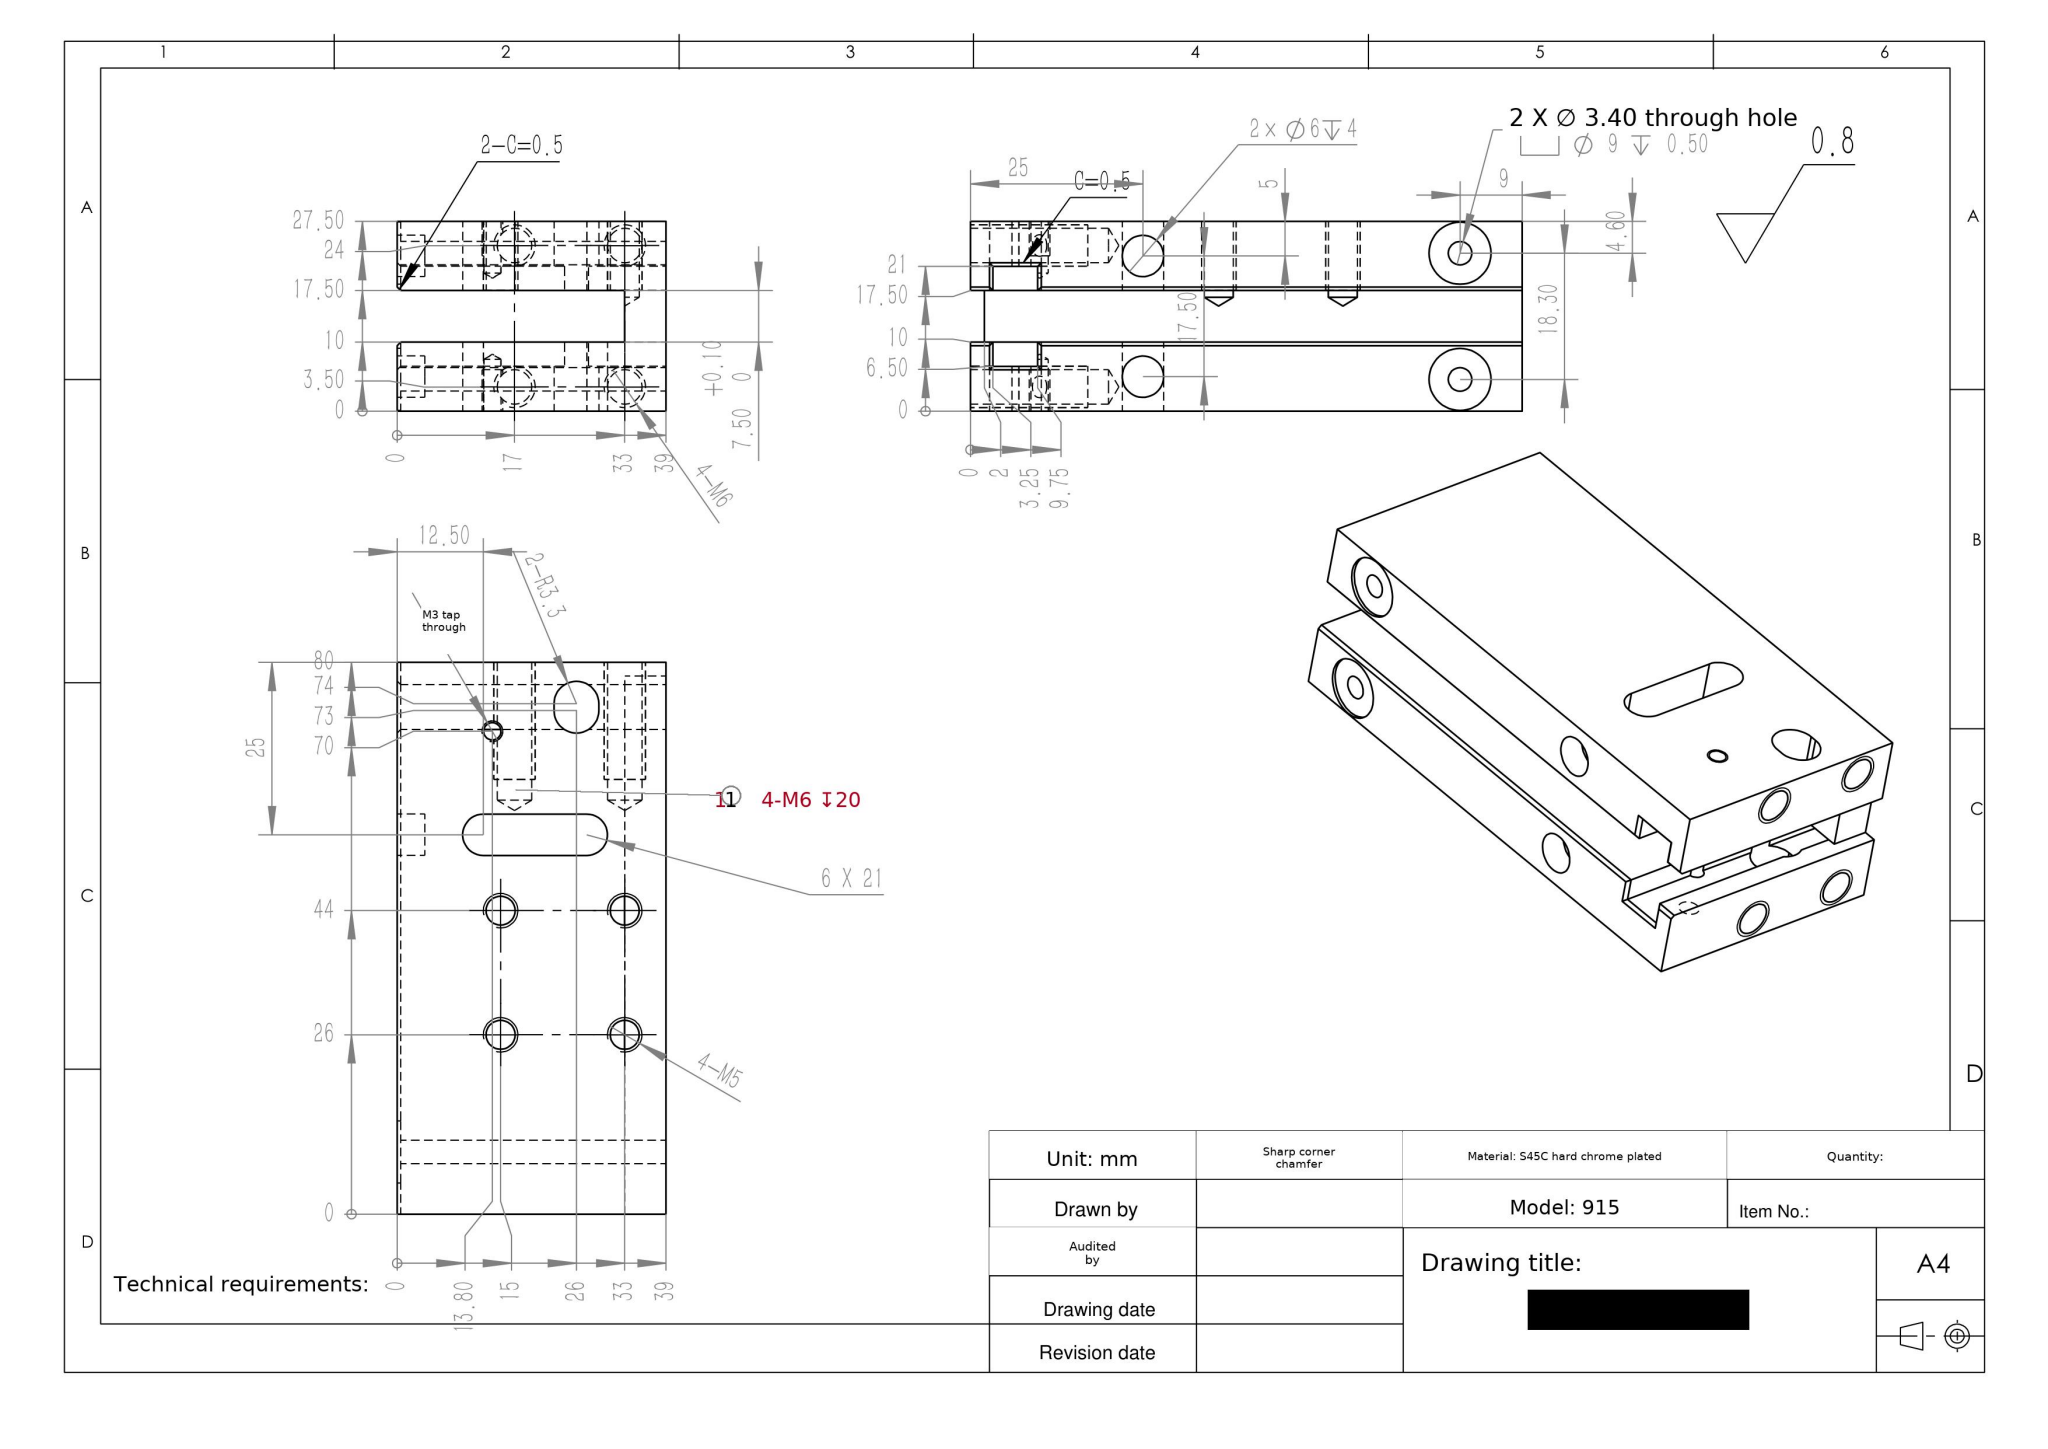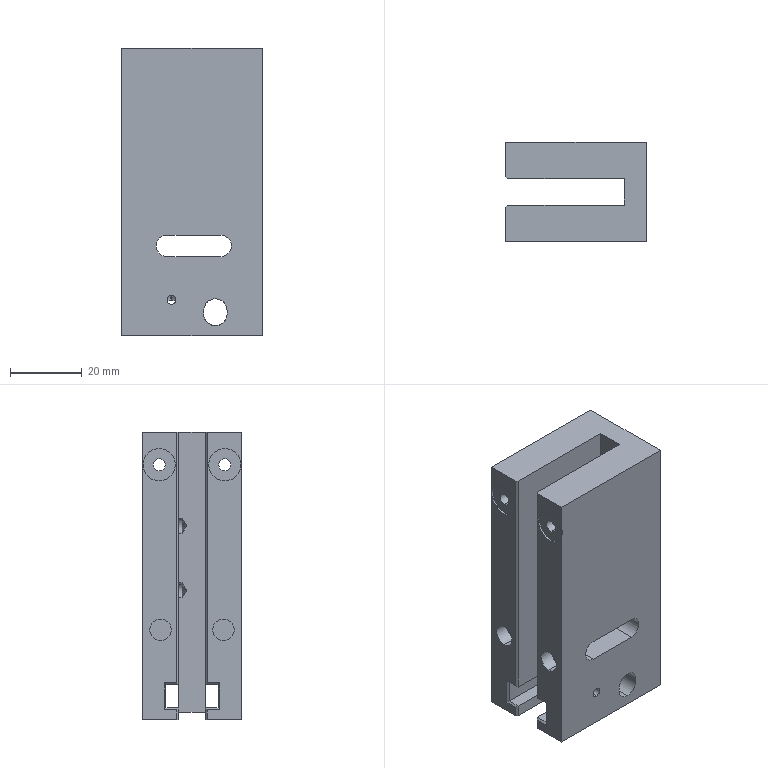Part | SolidWorks | mm | material S45C hard chrome plated | 1 solid | 106 faces | box 39 x 27.5 x 80 mm | volume 57974 mm3 | plane 50 | cylinder 42 | cone 14 | commonest cylinder face diameters 6 x8 5 x8 4.2 x8 6.5 x6 9 x4 3.4 x4 2.5 x4
build123d program:
from build123d import *

# Parameters (mm, degrees)
BOSS_EXTRUDE1_DEPTH                                 = 80
CHAMFER1_SIZE                                       = 0.5
SKETCH3_R                                           = 3.25
CUT_EXTRUDE1_DEPTH                                  = 94.152
SKETCH4_W                                           = 6.5
SKETCH4_H                                           = 3.5
CUT_EXTRUDE2_DEPTH                                  = 94.152
M5_TAPPED_HOLE1_D                                   = 4.2
M5_TAPPED_HOLE1_DEPTH                               = 11
M5_TAPPED_HOLE1_TIP                                 = 1.262
M6_TAPPED_HOLE1_D                                   = 5
M6_TAPPED_HOLE1_DEPTH                               = 20
M6_TAPPED_HOLE1_TIP                                 = 1.502
SKETCH8_W                                           = 6
SKETCH8_H                                           = 7.5
CUT_EXTRUDE3_DEPTH                                  = 2
CHAMFER2_SIZE                                       = 0.5
M3_TAPPED_HOLE1_D                                   = 2.5
M3_TAPPED_HOLE1_DEPTH                               = 7.5
M3_TAPPED_HOLE1_TIP                                 = 0.7511
M3_TAPPED_HOLE2_D                                   = 2.5
M3_TAPPED_HOLE2_DEPTH                               = 7.5
M3_TAPPED_HOLE2_TIP                                 = 0.7511
CUT_EXTRUDE4_DEPTH                                  = 94.152
CUT_EXTRUDE5_DEPTH                                  = 94.152
CYLINDRICAL_COUNTERSUNK_HOLE_FOR_M3_HEX_D           = 3.4
CYLINDRICAL_COUNTERSUNK_HOLE_FOR_M3_HEX_CBORE_D     = 9
CYLINDRICAL_COUNTERSUNK_HOLE_FOR_M3_HEX_CBORE_DEPTH = 0.5
SKETCH18_R                                          = 3
CUT_EXTRUDE6_DEPTH                                  = 4


with BuildPart() as part:
    # Sketch1 → Boss-Extrude1 (new body)
    with BuildSketch(Plane.XY):
        Polygon((0, 17.5), (0, 27.5), (39, 27.5), (39, 0), (0, 0), (0, 10), (33, 10), (33, 17.5), align=None)
    extrude(amount=BOSS_EXTRUDE1_DEPTH)

    # Chamfer1
    chamfer1_edges = [part.edges().sort_by_distance(p)[0] for p in [
        (0, 10, 40),
        (0, 17.5, 40),
    ]]
    chamfer(chamfer1_edges, length=CHAMFER1_SIZE)

    # Sketch3 → Cut-Extrude1 (cut, through all)
    with BuildSketch(Plane(origin=(0, 27.5, 0), x_dir=(1, 0, 0), z_dir=(0, 1, 0))):
        with Locations(Location((26, -6.5, 0), (0, 0, 270))):
            Circle(SKETCH3_R)
    extrude(amount=-CUT_EXTRUDE1_DEPTH, mode=Mode.SUBTRACT)

    # Sketch4 → Cut-Extrude2 (cut, through all)
    with BuildSketch(Plane.ZY):
        with Locations((6.5, 19.25)):
            Rectangle(SKETCH4_W, SKETCH4_H)
        with Locations((6.5, 8.25)):
            Rectangle(SKETCH4_W, SKETCH4_H)
    extrude(amount=-CUT_EXTRUDE2_DEPTH, mode=Mode.SUBTRACT)

    # M5 Tapped Hole1
    with Locations(Plane(origin=(15, 27.5, 36), x_dir=(0, 0, 1), z_dir=(0, 1, 0))):
        with Locations((0, 0), (0, 18), (18, 18), (18, 0)):
            Hole(M5_TAPPED_HOLE1_D / 2, depth=M5_TAPPED_HOLE1_DEPTH)
            with Locations((0, 0, -(M5_TAPPED_HOLE1_DEPTH + M5_TAPPED_HOLE1_TIP / 2))):  # 118° drill point
                Cone(0, M5_TAPPED_HOLE1_D / 2, M5_TAPPED_HOLE1_TIP, mode=Mode.SUBTRACT)

    # M6 Tapped Hole1
    with Locations(Plane(origin=(33, 24, 0), x_dir=(-1, 0, 0), z_dir=(0, 0, -1))):
        with Locations((0, 0), (16, 0), (16, -20.5), (0, -20.5)):
            Hole(M6_TAPPED_HOLE1_D / 2, depth=M6_TAPPED_HOLE1_DEPTH)
            with Locations((0, 0, -(M6_TAPPED_HOLE1_DEPTH + M6_TAPPED_HOLE1_TIP / 2))):  # 118° drill point
                Cone(0, M6_TAPPED_HOLE1_D / 2, M6_TAPPED_HOLE1_TIP, mode=Mode.SUBTRACT)

    # Sketch8 → Cut-Extrude3 (cut)
    with BuildSketch(Plane(origin=(0, 0, 0), x_dir=(-1, 0, 0), z_dir=(0, 0, -1))):
        with Locations((-36, 13.75)):
            Rectangle(SKETCH8_W, SKETCH8_H)
    extrude(amount=-CUT_EXTRUDE3_DEPTH, mode=Mode.SUBTRACT)

    # Chamfer2
    chamfer2_edges = [part.edges().sort_by_distance(p)[0] for p in [
        (0, 8, 3.25),
        (0, 8, 9.75),
        (0, 6.5, 6.5),
        (0, 19.5, 3.25),
        (0, 19.5, 9.75),
        (0, 21, 6.5),
    ]]
    chamfer(chamfer2_edges, length=CHAMFER2_SIZE)

    # M3 Tapped Hole1
    with Locations(Plane(origin=(13.8, 27.5, 10), x_dir=(0, 0, 1), z_dir=(0, 1, 0))):
        with Locations((0, 0)):
            Hole(M3_TAPPED_HOLE1_D / 2, depth=M3_TAPPED_HOLE1_DEPTH)
            with Locations((0, 0, -(M3_TAPPED_HOLE1_DEPTH + M3_TAPPED_HOLE1_TIP / 2))):  # 118° drill point
                Cone(0, M3_TAPPED_HOLE1_D / 2, M3_TAPPED_HOLE1_TIP, mode=Mode.SUBTRACT)

    # M3 Tapped Hole2
    with Locations(Plane(origin=(13.8, 0, 10), x_dir=(0, 0, -1), z_dir=(0, -1, 0))):
        with Locations((0, 0)):
            Hole(M3_TAPPED_HOLE2_D / 2, depth=M3_TAPPED_HOLE2_DEPTH)
            with Locations((0, 0, -(M3_TAPPED_HOLE2_DEPTH + M3_TAPPED_HOLE2_TIP / 2))):  # 118° drill point
                Cone(0, M3_TAPPED_HOLE2_D / 2, M3_TAPPED_HOLE2_TIP, mode=Mode.SUBTRACT)

    # Sketch12 → Cut-Extrude4 (cut, through all)
    with BuildSketch(Plane.XZ):
        with BuildLine():
            Line((29.25, 7), (29.25, 6))
            ThreePointArc((29.25, 6), (26, 2.75), (22.75, 6))
            Line((22.75, 6), (22.75, 7))
            ThreePointArc((22.75, 7), (26, 10.25), (29.25, 7))
        make_face()
    extrude(amount=-CUT_EXTRUDE4_DEPTH, mode=Mode.SUBTRACT)

    # Sketch13 → Cut-Extrude5 (cut, through all)
    with BuildSketch(Plane(origin=(0, 27.5, 0), x_dir=(1, 0, 0), z_dir=(0, 1, 0))):
        with BuildLine():
            Line((12.5, -22), (27.5, -22))
            ThreePointArc((27.5, -22), (30.5, -25), (27.5, -28))
            Line((27.5, -28), (12.5, -28))
            ThreePointArc((12.5, -28), (9.5, -25), (12.5, -22))
        make_face()
    extrude(amount=-CUT_EXTRUDE5_DEPTH, mode=Mode.SUBTRACT)

    # Cylindrical Countersunk Hole for M3 Hex (through all)
    with Locations(Plane.ZY):
        with Locations((71, 22.9), (71, 4.6)):
            CounterBoreHole(CYLINDRICAL_COUNTERSUNK_HOLE_FOR_M3_HEX_D / 2, CYLINDRICAL_COUNTERSUNK_HOLE_FOR_M3_HEX_CBORE_D / 2, CYLINDRICAL_COUNTERSUNK_HOLE_FOR_M3_HEX_CBORE_DEPTH)

    # Sketch18 → Cut-Extrude6 (cut)
    with BuildSketch(Plane.ZY):
        with Locations((25, 22.5)):
            Circle(SKETCH18_R)
        with Locations((25, 5)):
            Circle(SKETCH18_R)
    extrude(amount=-CUT_EXTRUDE6_DEPTH, mode=Mode.SUBTRACT)


solid = part.part